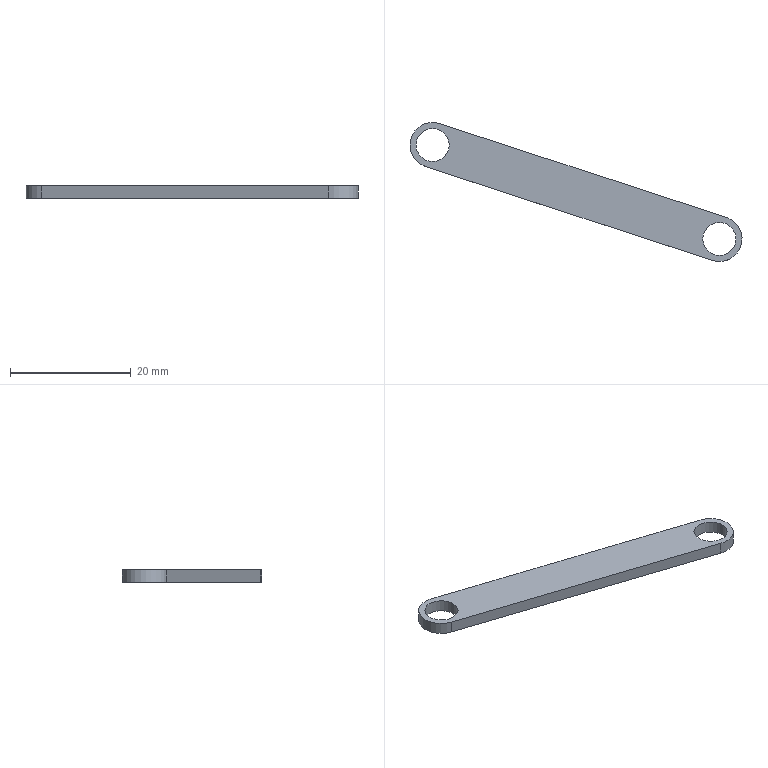Component | NX | CRANK_ROCKER_2 | 1 solid | 8 faces | box 55.02 x 23.05 x 2 mm | volume 743 mm3 | cylinder 4 | plane 4 | commonest cylinder face diameters 7.5 x2 5.5 x2
STEP:
#1=CARTESIAN_POINT('',(0.,0.,0.));
#2=DIRECTION('',(0.,0.,1.));
#3=DIRECTION('',(1.,0.,0.));
#4=AXIS2_PLACEMENT_3D('',#1,#2,#3);
#5=CARTESIAN_POINT('',(-8.947,10.249,-6.49));
#6=VERTEX_POINT('',#5);
#7=CARTESIAN_POINT('',(-11.28,3.121,-6.49));
#8=VERTEX_POINT('',#7);
#9=CARTESIAN_POINT('',(-10.114,6.685,-6.49));
#10=DIRECTION('',(0.,0.,1.));
#11=DIRECTION('',(0.9504,-0.3111,0.));
#12=AXIS2_PLACEMENT_3D('',#9,#10,#11);
#13=CIRCLE('',#12,3.75);
#14=CARTESIAN_POINT('',(-10.114,6.685,-4.49));
#15=DIRECTION('',(0.,0.,-1.));
#16=DIRECTION('',(-0.9504,0.3111,0.));
#17=AXIS2_PLACEMENT_3D('',#14,#15,#16);
#18=CYLINDRICAL_SURFACE('',#17,3.75);
#19=CARTESIAN_POINT('',(3.142,2.));
#20=DIRECTION('',(-1.,0.));
#21=VECTOR('',#20,1.);
#22=LINE('',#19,#21);
#23=(GEOMETRIC_REPRESENTATION_CONTEXT(2)PARAMETRIC_REPRESENTATION_CONTEXT()REPRESENTATION_CONTEXT('',''));
#24=DEFINITIONAL_REPRESENTATION('',(#22),#23);
#25=PCURVE('',#18,#24);
#26=CARTESIAN_POINT('',(-10.114,6.685,-6.49));
#27=DIRECTION('',(0.,0.,1.));
#28=DIRECTION('',(0.9504,-0.3111,0.));
#29=AXIS2_PLACEMENT_3D('',#26,#27,#28);
#30=PLANE('',#29);
#31=CARTESIAN_POINT('',(0.,0.));
#32=DIRECTION('',(1.,0.));
#33=AXIS2_PLACEMENT_2D('',#31,#32);
#34=CIRCLE('',#33,3.75);
#35=(GEOMETRIC_REPRESENTATION_CONTEXT(2)PARAMETRIC_REPRESENTATION_CONTEXT()REPRESENTATION_CONTEXT('',''));
#36=DEFINITIONAL_REPRESENTATION('',(#34),#35);
#37=PCURVE('',#30,#36);
#38=SURFACE_CURVE('',#13,(#25,#37),.PCURVE_S1.);
#39=EDGE_CURVE('',#6,#8,#38,.T.);
#40=ORIENTED_EDGE('',*,*,#39,.T.);
#41=CARTESIAN_POINT('',(-11.28,3.121,-4.49));
#42=VERTEX_POINT('',#41);
#43=CARTESIAN_POINT('',(-11.28,3.121,-4.49));
#44=DIRECTION('',(0.,0.,-1.));
#45=VECTOR('',#44,1.);
#46=LINE('',#43,#45);
#47=CARTESIAN_POINT('',(-1.571,0.));
#48=DIRECTION('',(0.,1.));
#49=VECTOR('',#48,1.);
#50=LINE('',#47,#49);
#51=(GEOMETRIC_REPRESENTATION_CONTEXT(2)PARAMETRIC_REPRESENTATION_CONTEXT()REPRESENTATION_CONTEXT('',''));
#52=DEFINITIONAL_REPRESENTATION('',(#50),#51);
#53=PCURVE('',#18,#52);
#54=CARTESIAN_POINT('',(-11.28,3.121,-4.49));
#55=DIRECTION('',(0.3111,0.9504,0.));
#56=DIRECTION('',(0.,0.,1.));
#57=AXIS2_PLACEMENT_3D('',#54,#55,#56);
#58=PLANE('',#57);
#59=CARTESIAN_POINT('',(0.,0.));
#60=DIRECTION('',(-1.,0.));
#61=VECTOR('',#60,1.);
#62=LINE('',#59,#61);
#63=(GEOMETRIC_REPRESENTATION_CONTEXT(2)PARAMETRIC_REPRESENTATION_CONTEXT()REPRESENTATION_CONTEXT('',''));
#64=DEFINITIONAL_REPRESENTATION('',(#62),#63);
#65=PCURVE('',#58,#64);
#66=SURFACE_CURVE('',#46,(#53,#65),.PCURVE_S1.);
#67=EDGE_CURVE('',#42,#8,#66,.T.);
#68=ORIENTED_EDGE('',*,*,#67,.F.);
#69=CARTESIAN_POINT('',(-8.947,10.249,-4.49));
#70=VERTEX_POINT('',#69);
#71=CARTESIAN_POINT('',(-10.114,6.685,-4.49));
#72=DIRECTION('',(0.,0.,1.));
#73=DIRECTION('',(0.9504,-0.3111,0.));
#74=AXIS2_PLACEMENT_3D('',#71,#72,#73);
#75=CIRCLE('',#74,3.75);
#76=CARTESIAN_POINT('',(3.142,0.));
#77=DIRECTION('',(-1.,0.));
#78=VECTOR('',#77,1.);
#79=LINE('',#76,#78);
#80=(GEOMETRIC_REPRESENTATION_CONTEXT(2)PARAMETRIC_REPRESENTATION_CONTEXT()REPRESENTATION_CONTEXT('',''));
#81=DEFINITIONAL_REPRESENTATION('',(#79),#80);
#82=PCURVE('',#18,#81);
#83=CARTESIAN_POINT('',(-10.114,6.685,-4.49));
#84=DIRECTION('',(0.,0.,1.));
#85=DIRECTION('',(0.9504,-0.3111,0.));
#86=AXIS2_PLACEMENT_3D('',#83,#84,#85);
#87=PLANE('',#86);
#88=CARTESIAN_POINT('',(0.,0.));
#89=DIRECTION('',(1.,0.));
#90=AXIS2_PLACEMENT_2D('',#88,#89);
#91=CIRCLE('',#90,3.75);
#92=(GEOMETRIC_REPRESENTATION_CONTEXT(2)PARAMETRIC_REPRESENTATION_CONTEXT()REPRESENTATION_CONTEXT('',''));
#93=DEFINITIONAL_REPRESENTATION('',(#91),#92);
#94=PCURVE('',#87,#93);
#95=SURFACE_CURVE('',#75,(#82,#94),.PCURVE_S1.);
#96=EDGE_CURVE('',#70,#42,#95,.T.);
#97=ORIENTED_EDGE('',*,*,#96,.F.);
#98=CARTESIAN_POINT('',(-8.947,10.249,-4.49));
#99=DIRECTION('',(0.,0.,-1.));
#100=VECTOR('',#99,1.);
#101=LINE('',#98,#100);
#102=CARTESIAN_POINT('',(1.571,0.));
#103=DIRECTION('',(0.,1.));
#104=VECTOR('',#103,1.);
#105=LINE('',#102,#104);
#106=(GEOMETRIC_REPRESENTATION_CONTEXT(2)PARAMETRIC_REPRESENTATION_CONTEXT()REPRESENTATION_CONTEXT('',''));
#107=DEFINITIONAL_REPRESENTATION('',(#105),#106);
#108=PCURVE('',#18,#107);
#109=CARTESIAN_POINT('',(38.572,-5.305,-4.49));
#110=DIRECTION('',(-0.3111,-0.9504,0.));
#111=DIRECTION('',(0.,0.,-1.));
#112=AXIS2_PLACEMENT_3D('',#109,#110,#111);
#113=PLANE('',#112);
#114=CARTESIAN_POINT('',(0.,-50.));
#115=DIRECTION('',(1.,0.));
#116=VECTOR('',#115,1.);
#117=LINE('',#114,#116);
#118=(GEOMETRIC_REPRESENTATION_CONTEXT(2)PARAMETRIC_REPRESENTATION_CONTEXT()REPRESENTATION_CONTEXT('',''));
#119=DEFINITIONAL_REPRESENTATION('',(#117),#118);
#120=PCURVE('',#113,#119);
#121=SURFACE_CURVE('',#101,(#108,#120),.PCURVE_S1.);
#122=EDGE_CURVE('',#70,#6,#121,.T.);
#123=ORIENTED_EDGE('',*,*,#122,.T.);
#124=EDGE_LOOP('',(#40,#68,#97,#123));
#125=FACE_BOUND('',#124,.T.);
#126=ADVANCED_FACE('',(#125),#18,.T.);
#127=CARTESIAN_POINT('',(36.239,-12.433,-6.49));
#128=VERTEX_POINT('',#127);
#129=CARTESIAN_POINT('',(-11.28,3.121,-6.49));
#130=DIRECTION('',(0.9504,-0.3111,0.));
#131=VECTOR('',#130,1.);
#132=LINE('',#129,#131);
#133=CARTESIAN_POINT('',(-2.,0.));
#134=DIRECTION('',(0.,1.));
#135=VECTOR('',#134,1.);
#136=LINE('',#133,#135);
#137=(GEOMETRIC_REPRESENTATION_CONTEXT(2)PARAMETRIC_REPRESENTATION_CONTEXT()REPRESENTATION_CONTEXT('',''));
#138=DEFINITIONAL_REPRESENTATION('',(#136),#137);
#139=PCURVE('',#58,#138);
#140=CARTESIAN_POINT('',(0.,-3.75));
#141=DIRECTION('',(1.,0.));
#142=VECTOR('',#141,1.);
#143=LINE('',#140,#142);
#144=(GEOMETRIC_REPRESENTATION_CONTEXT(2)PARAMETRIC_REPRESENTATION_CONTEXT()REPRESENTATION_CONTEXT('',''));
#145=DEFINITIONAL_REPRESENTATION('',(#143),#144);
#146=PCURVE('',#30,#145);
#147=SURFACE_CURVE('',#132,(#139,#146),.PCURVE_S1.);
#148=EDGE_CURVE('',#8,#128,#147,.T.);
#149=ORIENTED_EDGE('',*,*,#148,.T.);
#150=CARTESIAN_POINT('',(36.239,-12.433,-4.49));
#151=VERTEX_POINT('',#150);
#152=CARTESIAN_POINT('',(36.239,-12.433,-4.49));
#153=DIRECTION('',(0.,0.,-1.));
#154=VECTOR('',#153,1.);
#155=LINE('',#152,#154);
#156=CARTESIAN_POINT('',(0.,50.));
#157=DIRECTION('',(-1.,0.));
#158=VECTOR('',#157,1.);
#159=LINE('',#156,#158);
#160=(GEOMETRIC_REPRESENTATION_CONTEXT(2)PARAMETRIC_REPRESENTATION_CONTEXT()REPRESENTATION_CONTEXT('',''));
#161=DEFINITIONAL_REPRESENTATION('',(#159),#160);
#162=PCURVE('',#58,#161);
#163=CARTESIAN_POINT('',(37.406,-8.869,-4.49));
#164=DIRECTION('',(0.,0.,-1.));
#165=DIRECTION('',(-0.9504,0.3111,0.));
#166=AXIS2_PLACEMENT_3D('',#163,#164,#165);
#167=CYLINDRICAL_SURFACE('',#166,3.75);
#168=CARTESIAN_POINT('',(4.712,0.));
#169=DIRECTION('',(0.,1.));
#170=VECTOR('',#169,1.);
#171=LINE('',#168,#170);
#172=(GEOMETRIC_REPRESENTATION_CONTEXT(2)PARAMETRIC_REPRESENTATION_CONTEXT()REPRESENTATION_CONTEXT('',''));
#173=DEFINITIONAL_REPRESENTATION('',(#171),#172);
#174=PCURVE('',#167,#173);
#175=SURFACE_CURVE('',#155,(#162,#174),.PCURVE_S1.);
#176=EDGE_CURVE('',#151,#128,#175,.T.);
#177=ORIENTED_EDGE('',*,*,#176,.F.);
#178=CARTESIAN_POINT('',(-11.28,3.121,-4.49));
#179=DIRECTION('',(0.9504,-0.3111,0.));
#180=VECTOR('',#179,1.);
#181=LINE('',#178,#180);
#182=CARTESIAN_POINT('',(0.,0.));
#183=DIRECTION('',(0.,1.));
#184=VECTOR('',#183,1.);
#185=LINE('',#182,#184);
#186=(GEOMETRIC_REPRESENTATION_CONTEXT(2)PARAMETRIC_REPRESENTATION_CONTEXT()REPRESENTATION_CONTEXT('',''));
#187=DEFINITIONAL_REPRESENTATION('',(#185),#186);
#188=PCURVE('',#58,#187);
#189=CARTESIAN_POINT('',(0.,-3.75));
#190=DIRECTION('',(1.,0.));
#191=VECTOR('',#190,1.);
#192=LINE('',#189,#191);
#193=(GEOMETRIC_REPRESENTATION_CONTEXT(2)PARAMETRIC_REPRESENTATION_CONTEXT()REPRESENTATION_CONTEXT('',''));
#194=DEFINITIONAL_REPRESENTATION('',(#192),#193);
#195=PCURVE('',#87,#194);
#196=SURFACE_CURVE('',#181,(#188,#195),.PCURVE_S1.);
#197=EDGE_CURVE('',#42,#151,#196,.T.);
#198=ORIENTED_EDGE('',*,*,#197,.F.);
#199=ORIENTED_EDGE('',*,*,#67,.T.);
#200=EDGE_LOOP('',(#149,#177,#198,#199));
#201=FACE_BOUND('',#200,.T.);
#202=ADVANCED_FACE('',(#201),#58,.F.);
#203=CARTESIAN_POINT('',(38.572,-5.305,-6.49));
#204=VERTEX_POINT('',#203);
#205=CARTESIAN_POINT('',(37.406,-8.869,-6.49));
#206=DIRECTION('',(0.,0.,1.));
#207=DIRECTION('',(0.9504,-0.3111,0.));
#208=AXIS2_PLACEMENT_3D('',#205,#206,#207);
#209=CIRCLE('',#208,3.75);
#210=CARTESIAN_POINT('',(9.425,2.));
#211=DIRECTION('',(-1.,0.));
#212=VECTOR('',#211,1.);
#213=LINE('',#210,#212);
#214=(GEOMETRIC_REPRESENTATION_CONTEXT(2)PARAMETRIC_REPRESENTATION_CONTEXT()REPRESENTATION_CONTEXT('',''));
#215=DEFINITIONAL_REPRESENTATION('',(#213),#214);
#216=PCURVE('',#167,#215);
#217=CARTESIAN_POINT('',(50.,0.));
#218=DIRECTION('',(1.,0.));
#219=AXIS2_PLACEMENT_2D('',#217,#218);
#220=CIRCLE('',#219,3.75);
#221=(GEOMETRIC_REPRESENTATION_CONTEXT(2)PARAMETRIC_REPRESENTATION_CONTEXT()REPRESENTATION_CONTEXT('',''));
#222=DEFINITIONAL_REPRESENTATION('',(#220),#221);
#223=PCURVE('',#30,#222);
#224=SURFACE_CURVE('',#209,(#216,#223),.PCURVE_S1.);
#225=EDGE_CURVE('',#128,#204,#224,.T.);
#226=ORIENTED_EDGE('',*,*,#225,.T.);
#227=CARTESIAN_POINT('',(38.572,-5.305,-4.49));
#228=VERTEX_POINT('',#227);
#229=CARTESIAN_POINT('',(38.572,-5.305,-4.49));
#230=DIRECTION('',(0.,0.,-1.));
#231=VECTOR('',#230,1.);
#232=LINE('',#229,#231);
#233=CARTESIAN_POINT('',(1.571,0.));
#234=DIRECTION('',(0.,1.));
#235=VECTOR('',#234,1.);
#236=LINE('',#233,#235);
#237=(GEOMETRIC_REPRESENTATION_CONTEXT(2)PARAMETRIC_REPRESENTATION_CONTEXT()REPRESENTATION_CONTEXT('',''));
#238=DEFINITIONAL_REPRESENTATION('',(#236),#237);
#239=PCURVE('',#167,#238);
#240=CARTESIAN_POINT('',(0.,0.));
#241=DIRECTION('',(1.,0.));
#242=VECTOR('',#241,1.);
#243=LINE('',#240,#242);
#244=(GEOMETRIC_REPRESENTATION_CONTEXT(2)PARAMETRIC_REPRESENTATION_CONTEXT()REPRESENTATION_CONTEXT('',''));
#245=DEFINITIONAL_REPRESENTATION('',(#243),#244);
#246=PCURVE('',#113,#245);
#247=SURFACE_CURVE('',#232,(#239,#246),.PCURVE_S1.);
#248=EDGE_CURVE('',#228,#204,#247,.T.);
#249=ORIENTED_EDGE('',*,*,#248,.F.);
#250=CARTESIAN_POINT('',(37.406,-8.869,-4.49));
#251=DIRECTION('',(0.,0.,1.));
#252=DIRECTION('',(0.9504,-0.3111,0.));
#253=AXIS2_PLACEMENT_3D('',#250,#251,#252);
#254=CIRCLE('',#253,3.75);
#255=CARTESIAN_POINT('',(9.425,0.));
#256=DIRECTION('',(-1.,0.));
#257=VECTOR('',#256,1.);
#258=LINE('',#255,#257);
#259=(GEOMETRIC_REPRESENTATION_CONTEXT(2)PARAMETRIC_REPRESENTATION_CONTEXT()REPRESENTATION_CONTEXT('',''));
#260=DEFINITIONAL_REPRESENTATION('',(#258),#259);
#261=PCURVE('',#167,#260);
#262=CARTESIAN_POINT('',(50.,0.));
#263=DIRECTION('',(1.,0.));
#264=AXIS2_PLACEMENT_2D('',#262,#263);
#265=CIRCLE('',#264,3.75);
#266=(GEOMETRIC_REPRESENTATION_CONTEXT(2)PARAMETRIC_REPRESENTATION_CONTEXT()REPRESENTATION_CONTEXT('',''));
#267=DEFINITIONAL_REPRESENTATION('',(#265),#266);
#268=PCURVE('',#87,#267);
#269=SURFACE_CURVE('',#254,(#261,#268),.PCURVE_S1.);
#270=EDGE_CURVE('',#151,#228,#269,.T.);
#271=ORIENTED_EDGE('',*,*,#270,.F.);
#272=ORIENTED_EDGE('',*,*,#176,.T.);
#273=EDGE_LOOP('',(#226,#249,#271,#272));
#274=FACE_BOUND('',#273,.T.);
#275=ADVANCED_FACE('',(#274),#167,.T.);
#276=CARTESIAN_POINT('',(-7.5,5.829,-4.49));
#277=VERTEX_POINT('',#276);
#278=CARTESIAN_POINT('',(-10.114,6.685,-4.49));
#279=DIRECTION('',(0.,0.,1.));
#280=DIRECTION('',(0.9504,-0.3111,0.));
#281=AXIS2_PLACEMENT_3D('',#278,#279,#280);
#282=CIRCLE('',#281,2.75);
#283=CARTESIAN_POINT('',(-10.114,6.685,-4.49));
#284=DIRECTION('',(0.,0.,-1.));
#285=DIRECTION('',(-0.9504,0.3111,0.));
#286=AXIS2_PLACEMENT_3D('',#283,#284,#285);
#287=CYLINDRICAL_SURFACE('',#286,2.75);
#288=CARTESIAN_POINT('',(9.425,0.));
#289=DIRECTION('',(-1.,0.));
#290=VECTOR('',#289,1.);
#291=LINE('',#288,#290);
#292=(GEOMETRIC_REPRESENTATION_CONTEXT(2)PARAMETRIC_REPRESENTATION_CONTEXT()REPRESENTATION_CONTEXT('',''));
#293=DEFINITIONAL_REPRESENTATION('',(#291),#292);
#294=PCURVE('',#287,#293);
#295=CARTESIAN_POINT('',(0.,0.));
#296=DIRECTION('',(1.,0.));
#297=AXIS2_PLACEMENT_2D('',#295,#296);
#298=CIRCLE('',#297,2.75);
#299=(GEOMETRIC_REPRESENTATION_CONTEXT(2)PARAMETRIC_REPRESENTATION_CONTEXT()REPRESENTATION_CONTEXT('',''));
#300=DEFINITIONAL_REPRESENTATION('',(#298),#299);
#301=PCURVE('',#87,#300);
#302=SURFACE_CURVE('',#282,(#294,#301),.PCURVE_S1.);
#303=EDGE_CURVE('',#277,#277,#302,.T.);
#304=ORIENTED_EDGE('',*,*,#303,.F.);
#305=CARTESIAN_POINT('',(-7.5,5.829,-6.49));
#306=VERTEX_POINT('',#305);
#307=CARTESIAN_POINT('',(-7.5,5.829,-4.49));
#308=CARTESIAN_POINT('',(-7.5,5.829,-6.49));
#309=B_SPLINE_CURVE_WITH_KNOTS('',1,(#307,#308),.UNSPECIFIED.,.F.,.F.,(2,2),(0.,2.),.PIECEWISE_BEZIER_KNOTS.);
#310=CARTESIAN_POINT('',(9.425,0.));
#311=DIRECTION('',(0.,1.));
#312=VECTOR('',#311,1.);
#313=LINE('',#310,#312);
#314=(GEOMETRIC_REPRESENTATION_CONTEXT(2)PARAMETRIC_REPRESENTATION_CONTEXT()REPRESENTATION_CONTEXT('',''));
#315=DEFINITIONAL_REPRESENTATION('',(#313),#314);
#316=PCURVE('',#287,#315);
#317=CARTESIAN_POINT('',(3.142,0.));
#318=DIRECTION('',(0.,1.));
#319=VECTOR('',#318,1.);
#320=LINE('',#317,#319);
#321=(GEOMETRIC_REPRESENTATION_CONTEXT(2)PARAMETRIC_REPRESENTATION_CONTEXT()REPRESENTATION_CONTEXT('',''));
#322=DEFINITIONAL_REPRESENTATION('',(#320),#321);
#323=PCURVE('',#287,#322);
#324=SEAM_CURVE('',#309,(#316,#323),.PCURVE_S1.);
#325=EDGE_CURVE('',#277,#306,#324,.T.);
#326=ORIENTED_EDGE('',*,*,#325,.T.);
#327=CARTESIAN_POINT('',(-10.114,6.685,-6.49));
#328=DIRECTION('',(0.,0.,1.));
#329=DIRECTION('',(0.9504,-0.3111,0.));
#330=AXIS2_PLACEMENT_3D('',#327,#328,#329);
#331=CIRCLE('',#330,2.75);
#332=CARTESIAN_POINT('',(9.425,2.));
#333=DIRECTION('',(-1.,0.));
#334=VECTOR('',#333,1.);
#335=LINE('',#332,#334);
#336=(GEOMETRIC_REPRESENTATION_CONTEXT(2)PARAMETRIC_REPRESENTATION_CONTEXT()REPRESENTATION_CONTEXT('',''));
#337=DEFINITIONAL_REPRESENTATION('',(#335),#336);
#338=PCURVE('',#287,#337);
#339=CARTESIAN_POINT('',(0.,0.));
#340=DIRECTION('',(1.,0.));
#341=AXIS2_PLACEMENT_2D('',#339,#340);
#342=CIRCLE('',#341,2.75);
#343=(GEOMETRIC_REPRESENTATION_CONTEXT(2)PARAMETRIC_REPRESENTATION_CONTEXT()REPRESENTATION_CONTEXT('',''));
#344=DEFINITIONAL_REPRESENTATION('',(#342),#343);
#345=PCURVE('',#30,#344);
#346=SURFACE_CURVE('',#331,(#338,#345),.PCURVE_S1.);
#347=EDGE_CURVE('',#306,#306,#346,.T.);
#348=ORIENTED_EDGE('',*,*,#347,.T.);
#349=ORIENTED_EDGE('',*,*,#325,.F.);
#350=EDGE_LOOP('',(#304,#326,#348,#349));
#351=FACE_BOUND('',#350,.F.);
#352=ADVANCED_FACE('',(#351),#287,.F.);
#353=CARTESIAN_POINT('',(38.572,-5.305,-6.49));
#354=DIRECTION('',(-0.9504,0.3111,0.));
#355=VECTOR('',#354,1.);
#356=LINE('',#353,#355);
#357=CARTESIAN_POINT('',(2.,0.));
#358=DIRECTION('',(0.,-1.));
#359=VECTOR('',#358,1.);
#360=LINE('',#357,#359);
#361=(GEOMETRIC_REPRESENTATION_CONTEXT(2)PARAMETRIC_REPRESENTATION_CONTEXT()REPRESENTATION_CONTEXT('',''));
#362=DEFINITIONAL_REPRESENTATION('',(#360),#361);
#363=PCURVE('',#113,#362);
#364=CARTESIAN_POINT('',(50.,3.75));
#365=DIRECTION('',(-1.,0.));
#366=VECTOR('',#365,1.);
#367=LINE('',#364,#366);
#368=(GEOMETRIC_REPRESENTATION_CONTEXT(2)PARAMETRIC_REPRESENTATION_CONTEXT()REPRESENTATION_CONTEXT('',''));
#369=DEFINITIONAL_REPRESENTATION('',(#367),#368);
#370=PCURVE('',#30,#369);
#371=SURFACE_CURVE('',#356,(#363,#370),.PCURVE_S1.);
#372=EDGE_CURVE('',#204,#6,#371,.T.);
#373=ORIENTED_EDGE('',*,*,#372,.T.);
#374=ORIENTED_EDGE('',*,*,#122,.F.);
#375=CARTESIAN_POINT('',(38.572,-5.305,-4.49));
#376=DIRECTION('',(-0.9504,0.3111,0.));
#377=VECTOR('',#376,1.);
#378=LINE('',#375,#377);
#379=CARTESIAN_POINT('',(0.,0.));
#380=DIRECTION('',(0.,-1.));
#381=VECTOR('',#380,1.);
#382=LINE('',#379,#381);
#383=(GEOMETRIC_REPRESENTATION_CONTEXT(2)PARAMETRIC_REPRESENTATION_CONTEXT()REPRESENTATION_CONTEXT('',''));
#384=DEFINITIONAL_REPRESENTATION('',(#382),#383);
#385=PCURVE('',#113,#384);
#386=CARTESIAN_POINT('',(50.,3.75));
#387=DIRECTION('',(-1.,0.));
#388=VECTOR('',#387,1.);
#389=LINE('',#386,#388);
#390=(GEOMETRIC_REPRESENTATION_CONTEXT(2)PARAMETRIC_REPRESENTATION_CONTEXT()REPRESENTATION_CONTEXT('',''));
#391=DEFINITIONAL_REPRESENTATION('',(#389),#390);
#392=PCURVE('',#87,#391);
#393=SURFACE_CURVE('',#378,(#385,#392),.PCURVE_S1.);
#394=EDGE_CURVE('',#228,#70,#393,.T.);
#395=ORIENTED_EDGE('',*,*,#394,.F.);
#396=ORIENTED_EDGE('',*,*,#248,.T.);
#397=EDGE_LOOP('',(#373,#374,#395,#396));
#398=FACE_BOUND('',#397,.T.);
#399=ADVANCED_FACE('',(#398),#113,.F.);
#400=CARTESIAN_POINT('',(40.019,-9.724,-4.49));
#401=VERTEX_POINT('',#400);
#402=CARTESIAN_POINT('',(37.406,-8.869,-4.49));
#403=DIRECTION('',(0.,0.,1.));
#404=DIRECTION('',(0.9504,-0.3111,0.));
#405=AXIS2_PLACEMENT_3D('',#402,#403,#404);
#406=CIRCLE('',#405,2.75);
#407=CARTESIAN_POINT('',(37.406,-8.869,-4.49));
#408=DIRECTION('',(0.,0.,-1.));
#409=DIRECTION('',(-0.9504,0.3111,0.));
#410=AXIS2_PLACEMENT_3D('',#407,#408,#409);
#411=CYLINDRICAL_SURFACE('',#410,2.75);
#412=CARTESIAN_POINT('',(9.425,0.));
#413=DIRECTION('',(-1.,0.));
#414=VECTOR('',#413,1.);
#415=LINE('',#412,#414);
#416=(GEOMETRIC_REPRESENTATION_CONTEXT(2)PARAMETRIC_REPRESENTATION_CONTEXT()REPRESENTATION_CONTEXT('',''));
#417=DEFINITIONAL_REPRESENTATION('',(#415),#416);
#418=PCURVE('',#411,#417);
#419=CARTESIAN_POINT('',(50.,0.));
#420=DIRECTION('',(1.,0.));
#421=AXIS2_PLACEMENT_2D('',#419,#420);
#422=CIRCLE('',#421,2.75);
#423=(GEOMETRIC_REPRESENTATION_CONTEXT(2)PARAMETRIC_REPRESENTATION_CONTEXT()REPRESENTATION_CONTEXT('',''));
#424=DEFINITIONAL_REPRESENTATION('',(#422),#423);
#425=PCURVE('',#87,#424);
#426=SURFACE_CURVE('',#406,(#418,#425),.PCURVE_S1.);
#427=EDGE_CURVE('',#401,#401,#426,.T.);
#428=ORIENTED_EDGE('',*,*,#427,.F.);
#429=CARTESIAN_POINT('',(40.019,-9.724,-6.49));
#430=VERTEX_POINT('',#429);
#431=CARTESIAN_POINT('',(40.019,-9.724,-4.49));
#432=CARTESIAN_POINT('',(40.019,-9.724,-6.49));
#433=B_SPLINE_CURVE_WITH_KNOTS('',1,(#431,#432),.UNSPECIFIED.,.F.,.F.,(2,2),(0.,2.),.PIECEWISE_BEZIER_KNOTS.);
#434=CARTESIAN_POINT('',(9.425,0.));
#435=DIRECTION('',(0.,1.));
#436=VECTOR('',#435,1.);
#437=LINE('',#434,#436);
#438=(GEOMETRIC_REPRESENTATION_CONTEXT(2)PARAMETRIC_REPRESENTATION_CONTEXT()REPRESENTATION_CONTEXT('',''));
#439=DEFINITIONAL_REPRESENTATION('',(#437),#438);
#440=PCURVE('',#411,#439);
#441=CARTESIAN_POINT('',(3.142,0.));
#442=DIRECTION('',(0.,1.));
#443=VECTOR('',#442,1.);
#444=LINE('',#441,#443);
#445=(GEOMETRIC_REPRESENTATION_CONTEXT(2)PARAMETRIC_REPRESENTATION_CONTEXT()REPRESENTATION_CONTEXT('',''));
#446=DEFINITIONAL_REPRESENTATION('',(#444),#445);
#447=PCURVE('',#411,#446);
#448=SEAM_CURVE('',#433,(#440,#447),.PCURVE_S1.);
#449=EDGE_CURVE('',#401,#430,#448,.T.);
#450=ORIENTED_EDGE('',*,*,#449,.T.);
#451=CARTESIAN_POINT('',(37.406,-8.869,-6.49));
#452=DIRECTION('',(0.,0.,1.));
#453=DIRECTION('',(0.9504,-0.3111,0.));
#454=AXIS2_PLACEMENT_3D('',#451,#452,#453);
#455=CIRCLE('',#454,2.75);
#456=CARTESIAN_POINT('',(9.425,2.));
#457=DIRECTION('',(-1.,0.));
#458=VECTOR('',#457,1.);
#459=LINE('',#456,#458);
#460=(GEOMETRIC_REPRESENTATION_CONTEXT(2)PARAMETRIC_REPRESENTATION_CONTEXT()REPRESENTATION_CONTEXT('',''));
#461=DEFINITIONAL_REPRESENTATION('',(#459),#460);
#462=PCURVE('',#411,#461);
#463=CARTESIAN_POINT('',(50.,0.));
#464=DIRECTION('',(1.,0.));
#465=AXIS2_PLACEMENT_2D('',#463,#464);
#466=CIRCLE('',#465,2.75);
#467=(GEOMETRIC_REPRESENTATION_CONTEXT(2)PARAMETRIC_REPRESENTATION_CONTEXT()REPRESENTATION_CONTEXT('',''));
#468=DEFINITIONAL_REPRESENTATION('',(#466),#467);
#469=PCURVE('',#30,#468);
#470=SURFACE_CURVE('',#455,(#462,#469),.PCURVE_S1.);
#471=EDGE_CURVE('',#430,#430,#470,.T.);
#472=ORIENTED_EDGE('',*,*,#471,.T.);
#473=ORIENTED_EDGE('',*,*,#449,.F.);
#474=EDGE_LOOP('',(#428,#450,#472,#473));
#475=FACE_BOUND('',#474,.F.);
#476=ADVANCED_FACE('',(#475),#411,.F.);
#477=ORIENTED_EDGE('',*,*,#96,.T.);
#478=ORIENTED_EDGE('',*,*,#197,.T.);
#479=ORIENTED_EDGE('',*,*,#270,.T.);
#480=ORIENTED_EDGE('',*,*,#394,.T.);
#481=EDGE_LOOP('',(#477,#478,#479,#480));
#482=FACE_BOUND('',#481,.T.);
#483=ORIENTED_EDGE('',*,*,#303,.F.);
#484=EDGE_LOOP('',(#483));
#485=FACE_BOUND('',#484,.T.);
#486=ORIENTED_EDGE('',*,*,#427,.F.);
#487=EDGE_LOOP('',(#486));
#488=FACE_BOUND('',#487,.T.);
#489=ADVANCED_FACE('',(#482,#485,#488),#87,.T.);
#490=ORIENTED_EDGE('',*,*,#39,.F.);
#491=ORIENTED_EDGE('',*,*,#372,.F.);
#492=ORIENTED_EDGE('',*,*,#225,.F.);
#493=ORIENTED_EDGE('',*,*,#148,.F.);
#494=EDGE_LOOP('',(#490,#491,#492,#493));
#495=FACE_BOUND('',#494,.T.);
#496=ORIENTED_EDGE('',*,*,#347,.T.);
#497=EDGE_LOOP('',(#496));
#498=FACE_BOUND('',#497,.T.);
#499=ORIENTED_EDGE('',*,*,#471,.T.);
#500=EDGE_LOOP('',(#499));
#501=FACE_BOUND('',#500,.T.);
#502=ADVANCED_FACE('',(#495,#498,#501),#30,.F.);
#503=CLOSED_SHELL('',(#126,#202,#275,#352,#399,#476,#489,#502));
#504=MANIFOLD_SOLID_BREP('',#503);
#505=(LENGTH_UNIT()NAMED_UNIT(*)SI_UNIT(.MILLI.,.METRE.));
#506=UNCERTAINTY_MEASURE_WITH_UNIT(LENGTH_MEASURE(0.000002),#505,'','');
#507=(NAMED_UNIT(*)PLANE_ANGLE_UNIT()SI_UNIT($,.RADIAN.));
#508=(NAMED_UNIT(*)SI_UNIT($,.STERADIAN.)SOLID_ANGLE_UNIT());
#509=(GEOMETRIC_REPRESENTATION_CONTEXT(3)GLOBAL_UNCERTAINTY_ASSIGNED_CONTEXT((#506))GLOBAL_UNIT_ASSIGNED_CONTEXT((#505,#507,#508))REPRESENTATION_CONTEXT('',''));
#510=ADVANCED_BREP_SHAPE_REPRESENTATION('',(#4,#504),#509);